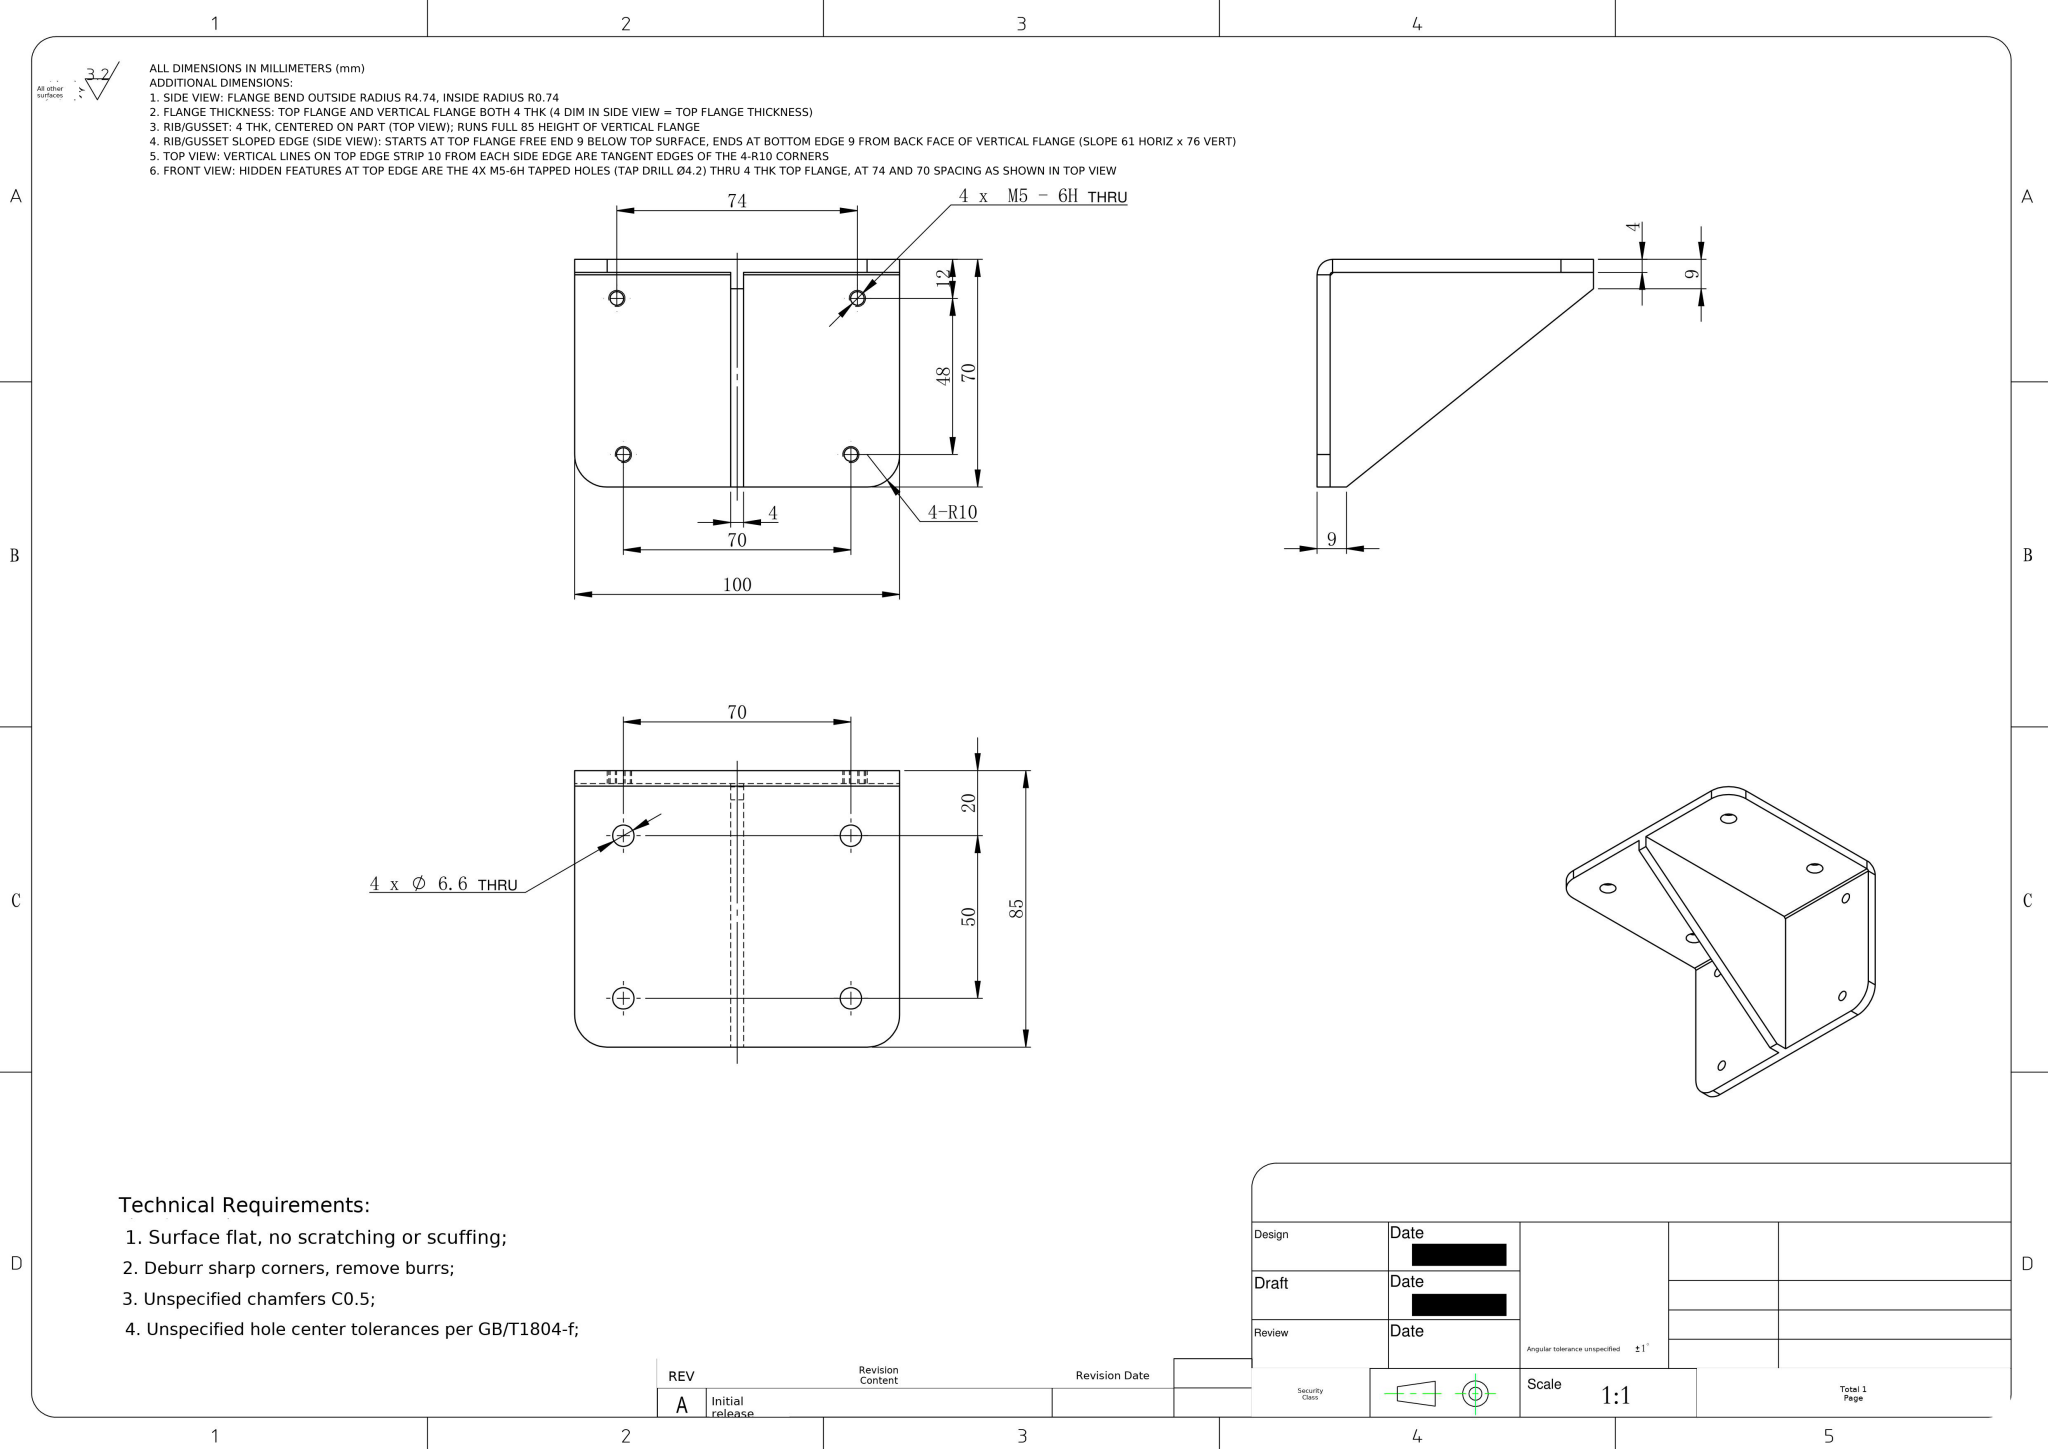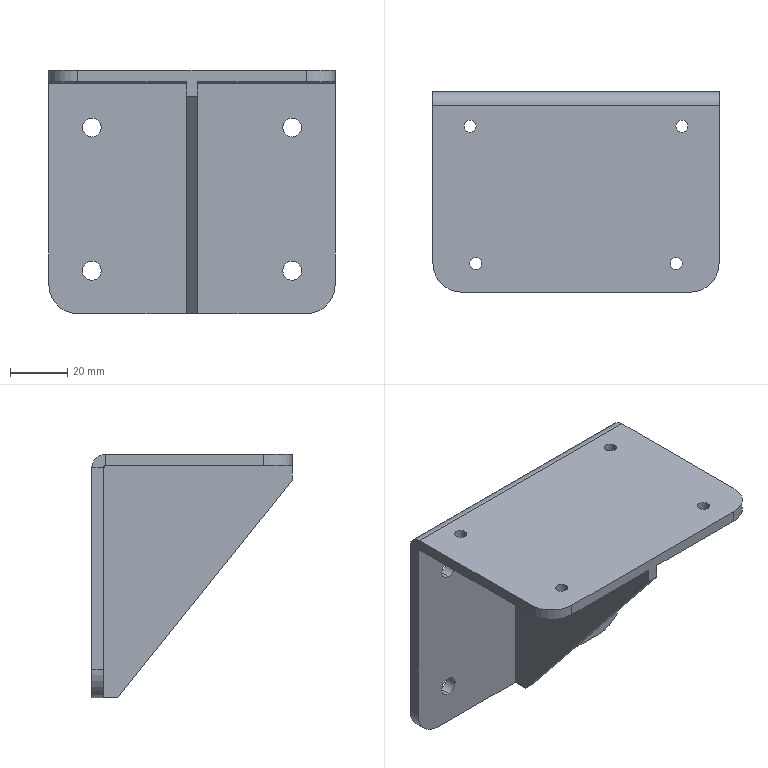Part | NX | mm | 1 solid | 38 faces | box 100 x 70 x 85 mm | volume 70928 mm3 | cylinder 22 | plane 16 | commonest cylinder face diameters 6.6 x8 4.2 x8 20 x4 9.473 x1 1.473 x1